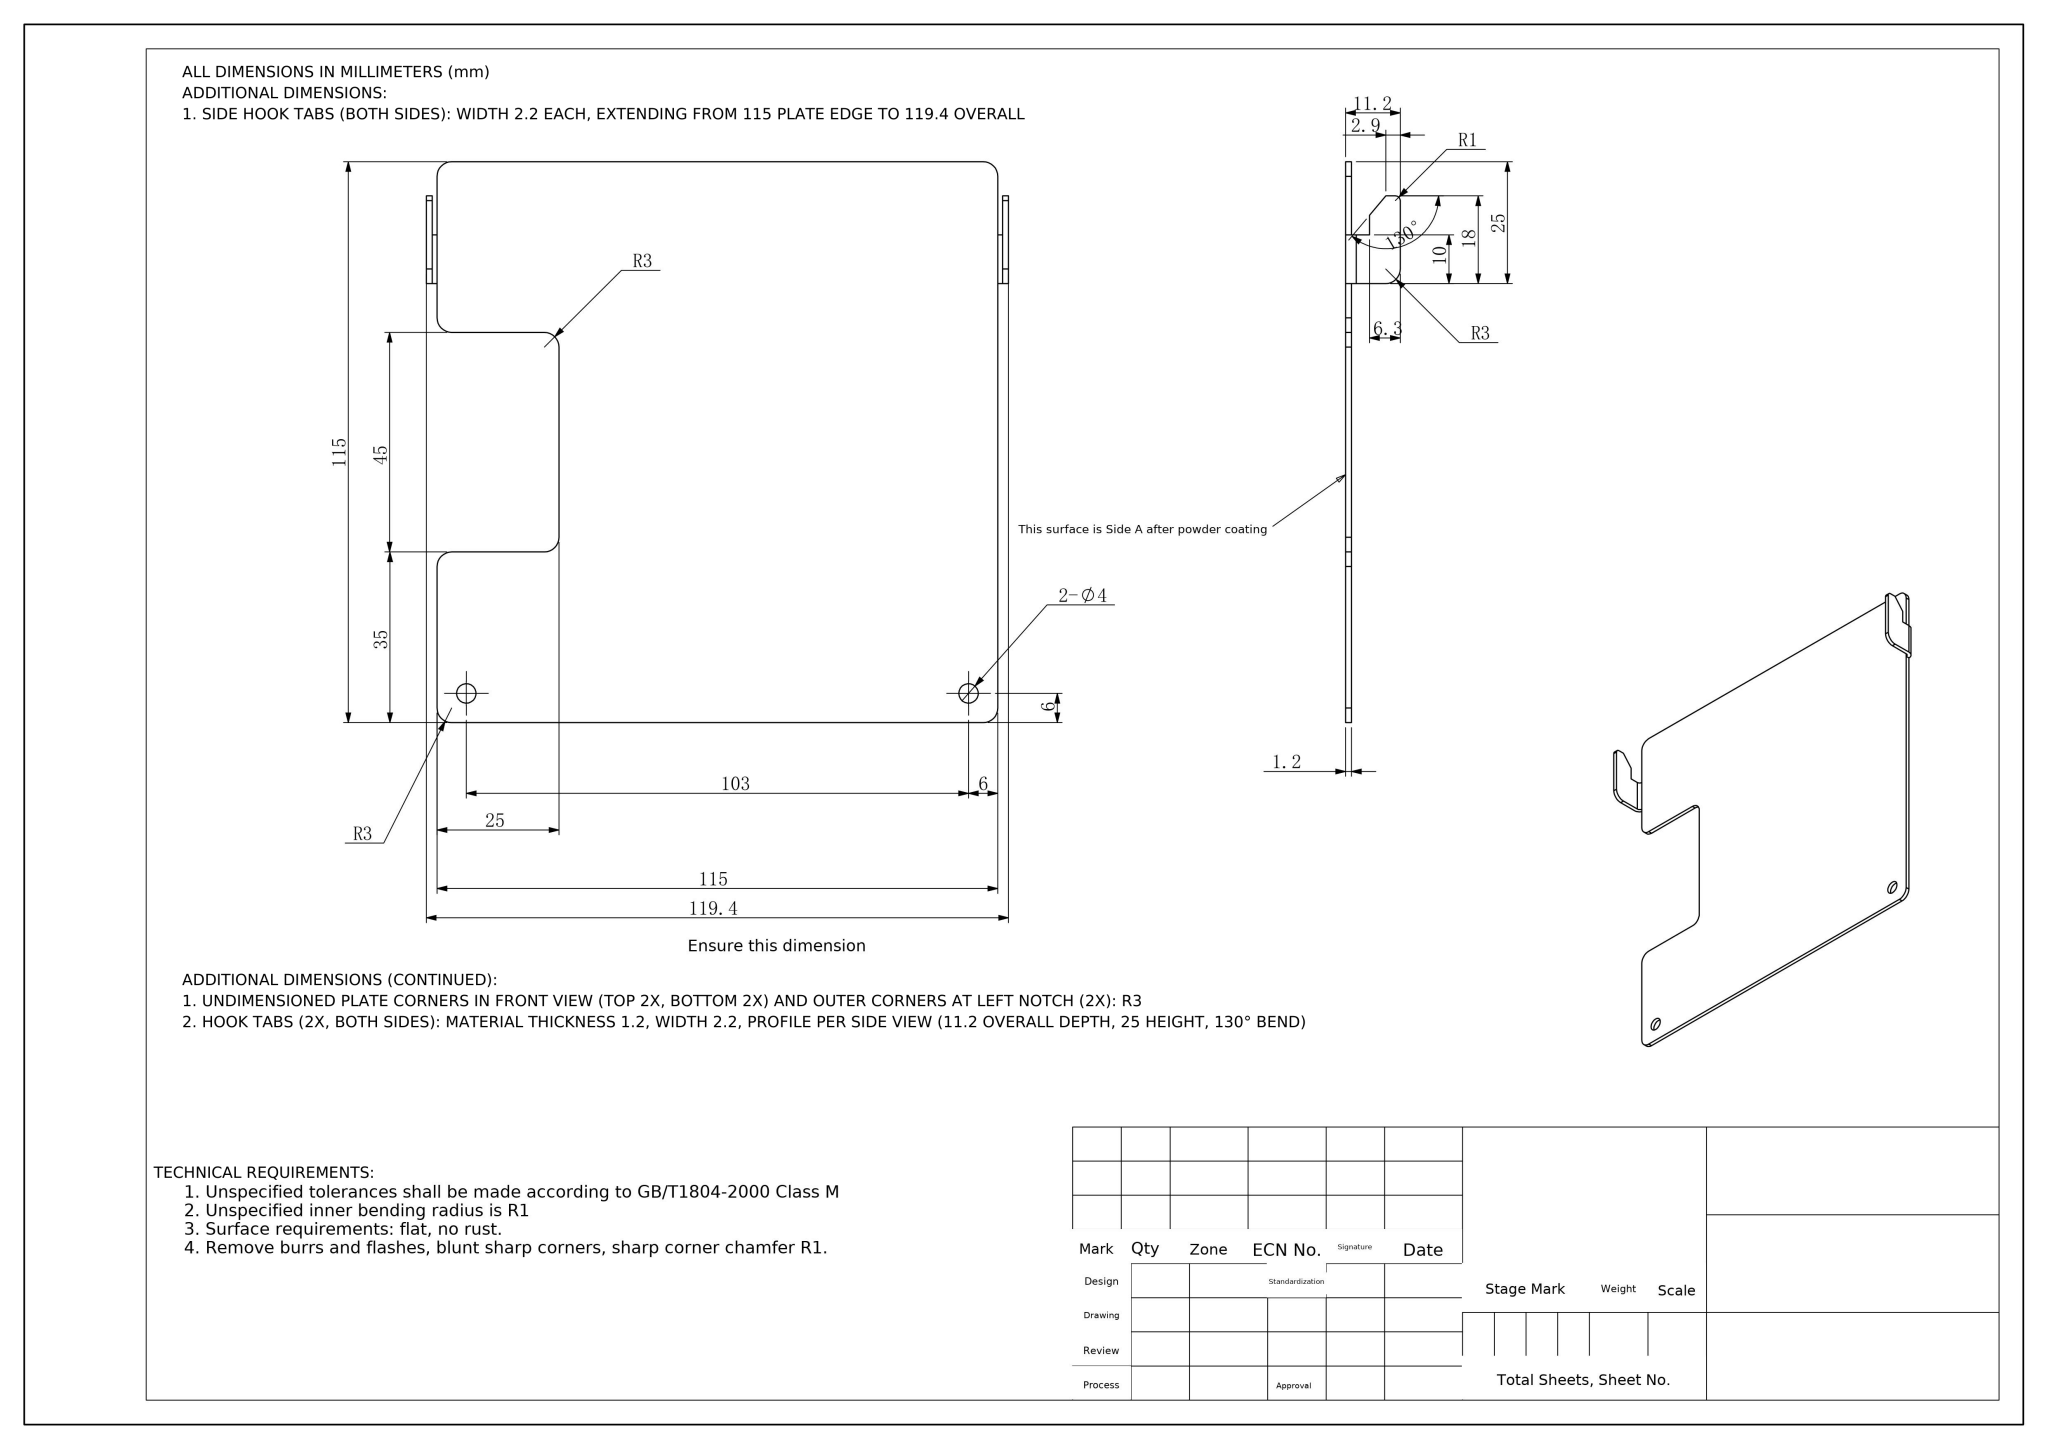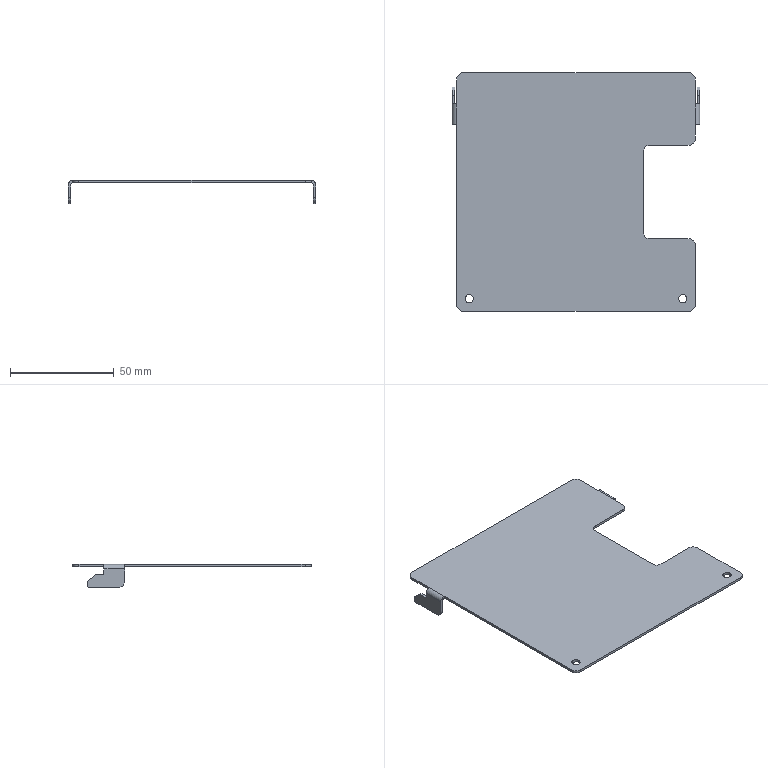Part | NX | mm | 1 solid | 48 faces | box 119.4 x 115 x 11.2 mm | volume 14857 mm3 | plane 28 | cylinder 20 | commonest cylinder face diameters 6 x10 4 x4 2 x4 4.4 x2